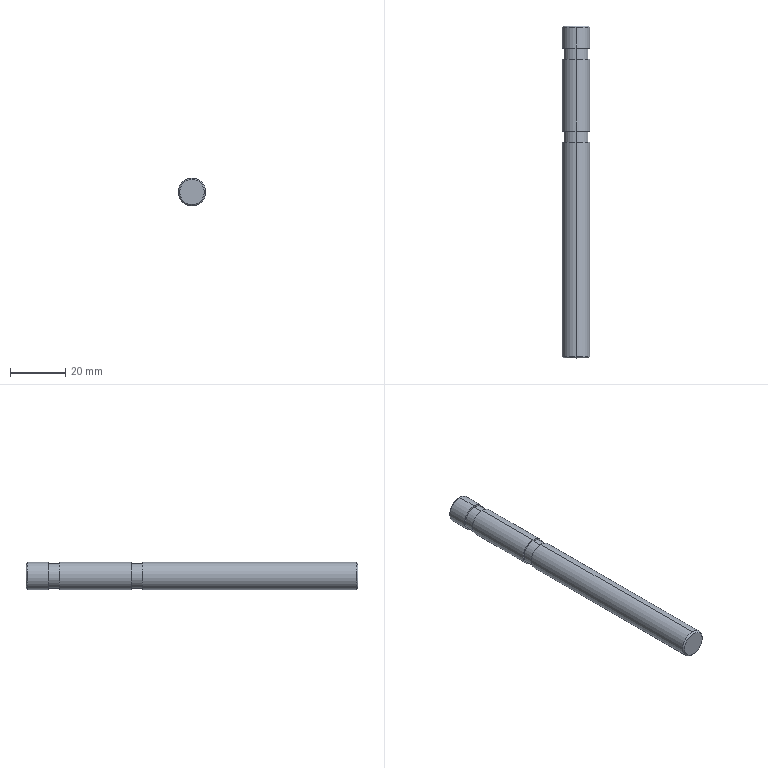Component | SolidWorks | 8TC-A15004-60-30A-2 | 1 solid | 20 faces | box 10 x 120 x 10 mm | volume 9298 mm3 | cylinder 10 | plane 6 | cone 4 | commonest cylinder face diameters 10 x6 9 x4 | material Chrome Plated Hard Rod
build123d program:
from build123d import *

# Parameters (mm, degrees)
SKETCH1_R           = 5
BOSS_EXTRUDE1_DEPTH = 60
CHAMFER1_SIZE       = 0.5
SKETCH2_W           = 1
SKETCH2_H           = 4


with BuildPart() as part:
    # Sketch1 → Boss-Extrude1 (new, symmetric)
    with BuildSketch(Plane(origin=(0, 0, 0), x_dir=(1, 0, 0), z_dir=(0, 1, 0))):
        with Locations(Location((0, 0, 0), (0, 0, 270))):
            Circle(SKETCH1_R)
    extrude(amount=BOSS_EXTRUDE1_DEPTH, both=True)

    # Chamfer1
    chamfer1_edges = [part.edges().sort_by_distance(p)[0] for p in [
        (0, -60, -5),
        (0, 60, -5),
    ]]
    chamfer(chamfer1_edges, length=CHAMFER1_SIZE)

    # Sketch2 → Cut-Revolve1 (revolve, cut)
    with BuildSketch(Plane.XY, mode=Mode.PRIVATE) as cut_revolve1_sk:
        with Locations((5, 50)):
            Rectangle(SKETCH2_W, SKETCH2_H)
        with Locations((5, 20)):
            Rectangle(SKETCH2_W, SKETCH2_H)
    revolve(cut_revolve1_sk.sketch.rotate(Axis((0, 0, 0), (0, -1, 0)), 90), axis=Axis((0, 0, 0), (0, -1, 0)), mode=Mode.SUBTRACT)


solid = part.part

# Placed as in the assembly
solid = solid.moved(Location((-88.286, -35, 0), (0, 0, 0)))
STEP:
#1=COLOUR_RGB('',0.7922,0.8196,0.9333);
#2=FILL_AREA_STYLE_COLOUR('',#1);
#3=FILL_AREA_STYLE('',(#2));
#4=SURFACE_STYLE_FILL_AREA(#3);
#5=SURFACE_SIDE_STYLE('',(#4));
#6=SURFACE_STYLE_USAGE(.BOTH.,#5);
#7=PRESENTATION_STYLE_ASSIGNMENT((#6));
#8=CARTESIAN_POINT('',(-3.476,-0.6693,0.1969));
#9=VERTEX_POINT('',#8);
#10=CARTESIAN_POINT('',(-3.476,-0.6693,-0.1969));
#11=VERTEX_POINT('',#10);
#12=CARTESIAN_POINT('',(-3.476,-0.6693,-0.));
#13=DIRECTION('',(0.,1.,0.));
#14=DIRECTION('',(0.,0.,1.));
#15=AXIS2_PLACEMENT_3D('',#12,#13,#14);
#16=CIRCLE('',#15,0.1969);
#17=EDGE_CURVE('',#9,#11,#16,.T.);
#18=ORIENTED_EDGE('',*,*,#17,.F.);
#19=CARTESIAN_POINT('',(-3.476,-3.72,0.1969));
#20=VERTEX_POINT('',#19);
#21=CARTESIAN_POINT('',(-3.476,0.9843,0.1969));
#22=DIRECTION('',(0.,-1.,0.));
#23=VECTOR('',#22,39.37);
#24=LINE('',#21,#23);
#25=EDGE_CURVE('',#9,#20,#24,.T.);
#26=ORIENTED_EDGE('',*,*,#25,.T.);
#27=CARTESIAN_POINT('',(-3.476,-3.72,-0.1969));
#28=VERTEX_POINT('',#27);
#29=CARTESIAN_POINT('',(-3.476,-3.72,-0.));
#30=DIRECTION('',(0.,1.,0.));
#31=DIRECTION('',(0.,0.,1.));
#32=AXIS2_PLACEMENT_3D('',#29,#30,#31);
#33=CIRCLE('',#32,0.1969);
#34=EDGE_CURVE('',#20,#28,#33,.T.);
#35=ORIENTED_EDGE('',*,*,#34,.T.);
#36=CARTESIAN_POINT('',(-3.476,0.9843,-0.1969));
#37=DIRECTION('',(0.,-1.,0.));
#38=VECTOR('',#37,39.37);
#39=LINE('',#36,#38);
#40=EDGE_CURVE('',#11,#28,#39,.T.);
#41=ORIENTED_EDGE('',*,*,#40,.F.);
#42=EDGE_LOOP('',(#18,#26,#35,#41));
#43=FACE_OUTER_BOUND('',#42,.T.);
#44=CARTESIAN_POINT('',(-3.476,0.9843,-0.));
#45=DIRECTION('',(0.,-1.,0.));
#46=DIRECTION('',(0.,0.,-1.));
#47=AXIS2_PLACEMENT_3D('',#44,#45,#46);
#48=CYLINDRICAL_SURFACE('',#47,0.1969);
#49=ADVANCED_FACE('',(#43),#48,.T.);
#50=CARTESIAN_POINT('',(-3.476,-3.74,-0.1772));
#51=VERTEX_POINT('',#50);
#52=CARTESIAN_POINT('',(-3.476,-3.74,0.1772));
#53=VERTEX_POINT('',#52);
#54=CARTESIAN_POINT('',(-3.476,-3.74,-0.));
#55=DIRECTION('',(0.,-1.,0.));
#56=DIRECTION('',(0.,0.,1.));
#57=AXIS2_PLACEMENT_3D('',#54,#55,#56);
#58=CIRCLE('',#57,0.1772);
#59=EDGE_CURVE('',#51,#53,#58,.T.);
#60=ORIENTED_EDGE('',*,*,#59,.F.);
#61=CARTESIAN_POINT('',(-3.476,-3.72,-0.1969));
#62=DIRECTION('',(0.,0.7071,-0.7071));
#63=VECTOR('',#62,39.37);
#64=LINE('',#61,#63);
#65=EDGE_CURVE('',#51,#28,#64,.T.);
#66=ORIENTED_EDGE('',*,*,#65,.T.);
#67=ORIENTED_EDGE('',*,*,#34,.F.);
#68=CARTESIAN_POINT('',(-3.476,-3.72,0.1969));
#69=DIRECTION('',(0.,0.7071,0.7071));
#70=VECTOR('',#69,39.37);
#71=LINE('',#68,#70);
#72=EDGE_CURVE('',#53,#20,#71,.T.);
#73=ORIENTED_EDGE('',*,*,#72,.F.);
#74=EDGE_LOOP('',(#60,#66,#67,#73));
#75=FACE_OUTER_BOUND('',#74,.T.);
#76=CARTESIAN_POINT('',(-3.476,-3.72,-0.));
#77=DIRECTION('',(0.,1.,0.));
#78=DIRECTION('',(0.,0.,1.));
#79=AXIS2_PLACEMENT_3D('',#76,#77,#78);
#80=CONICAL_SURFACE('',#79,0.1969,0.7854);
#81=ADVANCED_FACE('',(#75),#80,.T.);
#82=CARTESIAN_POINT('',(-3.476,-0.6693,0.1772));
#83=VERTEX_POINT('',#82);
#84=CARTESIAN_POINT('',(-3.476,-0.6693,-0.1772));
#85=VERTEX_POINT('',#84);
#86=CARTESIAN_POINT('',(-3.476,-0.6693,-0.));
#87=DIRECTION('',(0.,1.,0.));
#88=DIRECTION('',(0.,0.,1.));
#89=AXIS2_PLACEMENT_3D('',#86,#87,#88);
#90=CIRCLE('',#89,0.1772);
#91=EDGE_CURVE('',#83,#85,#90,.T.);
#92=ORIENTED_EDGE('',*,*,#91,.T.);
#93=CARTESIAN_POINT('',(-3.476,-0.5118,-0.1772));
#94=VERTEX_POINT('',#93);
#95=CARTESIAN_POINT('',(-3.476,-1.378,-0.1772));
#96=DIRECTION('',(0.,1.,0.));
#97=VECTOR('',#96,39.37);
#98=LINE('',#95,#97);
#99=EDGE_CURVE('',#85,#94,#98,.T.);
#100=ORIENTED_EDGE('',*,*,#99,.T.);
#101=CARTESIAN_POINT('',(-3.476,-0.5118,0.1772));
#102=VERTEX_POINT('',#101);
#103=CARTESIAN_POINT('',(-3.476,-0.5118,-0.));
#104=DIRECTION('',(0.,1.,0.));
#105=DIRECTION('',(0.,0.,1.));
#106=AXIS2_PLACEMENT_3D('',#103,#104,#105);
#107=CIRCLE('',#106,0.1772);
#108=EDGE_CURVE('',#102,#94,#107,.T.);
#109=ORIENTED_EDGE('',*,*,#108,.F.);
#110=CARTESIAN_POINT('',(-3.476,-1.378,0.1772));
#111=DIRECTION('',(0.,1.,0.));
#112=VECTOR('',#111,39.37);
#113=LINE('',#110,#112);
#114=EDGE_CURVE('',#83,#102,#113,.T.);
#115=ORIENTED_EDGE('',*,*,#114,.F.);
#116=EDGE_LOOP('',(#92,#100,#109,#115));
#117=FACE_OUTER_BOUND('',#116,.T.);
#118=CARTESIAN_POINT('',(-3.476,-1.378,-0.));
#119=DIRECTION('',(0.,1.,0.));
#120=DIRECTION('',(0.,0.,1.));
#121=AXIS2_PLACEMENT_3D('',#118,#119,#120);
#122=CYLINDRICAL_SURFACE('',#121,0.1772);
#123=ADVANCED_FACE('',(#117),#122,.T.);
#124=CARTESIAN_POINT('',(-3.476,0.5118,0.1772));
#125=VERTEX_POINT('',#124);
#126=CARTESIAN_POINT('',(-3.476,0.5118,-0.1772));
#127=VERTEX_POINT('',#126);
#128=CARTESIAN_POINT('',(-3.476,0.5118,-0.));
#129=DIRECTION('',(0.,1.,0.));
#130=DIRECTION('',(0.,0.,1.));
#131=AXIS2_PLACEMENT_3D('',#128,#129,#130);
#132=CIRCLE('',#131,0.1772);
#133=EDGE_CURVE('',#125,#127,#132,.T.);
#134=ORIENTED_EDGE('',*,*,#133,.T.);
#135=CARTESIAN_POINT('',(-3.476,0.6693,-0.1772));
#136=VERTEX_POINT('',#135);
#137=CARTESIAN_POINT('',(-3.476,-1.378,-0.1772));
#138=DIRECTION('',(0.,1.,0.));
#139=VECTOR('',#138,39.37);
#140=LINE('',#137,#139);
#141=EDGE_CURVE('',#127,#136,#140,.T.);
#142=ORIENTED_EDGE('',*,*,#141,.T.);
#143=CARTESIAN_POINT('',(-3.476,0.6693,0.1772));
#144=VERTEX_POINT('',#143);
#145=CARTESIAN_POINT('',(-3.476,0.6693,-0.));
#146=DIRECTION('',(0.,1.,0.));
#147=DIRECTION('',(0.,0.,1.));
#148=AXIS2_PLACEMENT_3D('',#145,#146,#147);
#149=CIRCLE('',#148,0.1772);
#150=EDGE_CURVE('',#144,#136,#149,.T.);
#151=ORIENTED_EDGE('',*,*,#150,.F.);
#152=CARTESIAN_POINT('',(-3.476,-1.378,0.1772));
#153=DIRECTION('',(0.,1.,0.));
#154=VECTOR('',#153,39.37);
#155=LINE('',#152,#154);
#156=EDGE_CURVE('',#125,#144,#155,.T.);
#157=ORIENTED_EDGE('',*,*,#156,.F.);
#158=EDGE_LOOP('',(#134,#142,#151,#157));
#159=FACE_OUTER_BOUND('',#158,.T.);
#160=CARTESIAN_POINT('',(-3.476,-1.378,-0.));
#161=DIRECTION('',(0.,1.,0.));
#162=DIRECTION('',(0.,0.,1.));
#163=AXIS2_PLACEMENT_3D('',#160,#161,#162);
#164=CYLINDRICAL_SURFACE('',#163,0.1772);
#165=ADVANCED_FACE('',(#159),#164,.T.);
#166=CARTESIAN_POINT('',(-3.476,0.9843,0.1772));
#167=VERTEX_POINT('',#166);
#168=CARTESIAN_POINT('',(-3.476,0.9843,-0.1772));
#169=VERTEX_POINT('',#168);
#170=CARTESIAN_POINT('',(-3.476,0.9843,-0.));
#171=DIRECTION('',(0.,1.,0.));
#172=DIRECTION('',(0.,0.,1.));
#173=AXIS2_PLACEMENT_3D('',#170,#171,#172);
#174=CIRCLE('',#173,0.1772);
#175=EDGE_CURVE('',#167,#169,#174,.T.);
#176=ORIENTED_EDGE('',*,*,#175,.F.);
#177=CARTESIAN_POINT('',(-3.476,0.9646,0.1969));
#178=VERTEX_POINT('',#177);
#179=CARTESIAN_POINT('',(-3.476,0.9843,0.1772));
#180=DIRECTION('',(0.,-0.7071,0.7071));
#181=VECTOR('',#180,39.37);
#182=LINE('',#179,#181);
#183=EDGE_CURVE('',#167,#178,#182,.T.);
#184=ORIENTED_EDGE('',*,*,#183,.T.);
#185=CARTESIAN_POINT('',(-3.476,0.9646,-0.1969));
#186=VERTEX_POINT('',#185);
#187=CARTESIAN_POINT('',(-3.476,0.9646,-0.));
#188=DIRECTION('',(0.,-1.,0.));
#189=DIRECTION('',(0.,0.,1.));
#190=AXIS2_PLACEMENT_3D('',#187,#188,#189);
#191=CIRCLE('',#190,0.1969);
#192=EDGE_CURVE('',#186,#178,#191,.T.);
#193=ORIENTED_EDGE('',*,*,#192,.F.);
#194=CARTESIAN_POINT('',(-3.476,0.9843,-0.1772));
#195=DIRECTION('',(0.,-0.7071,-0.7071));
#196=VECTOR('',#195,39.37);
#197=LINE('',#194,#196);
#198=EDGE_CURVE('',#169,#186,#197,.T.);
#199=ORIENTED_EDGE('',*,*,#198,.F.);
#200=EDGE_LOOP('',(#176,#184,#193,#199));
#201=FACE_OUTER_BOUND('',#200,.T.);
#202=CARTESIAN_POINT('',(-3.476,0.9843,-0.));
#203=DIRECTION('',(0.,-1.,0.));
#204=DIRECTION('',(0.,0.,-1.));
#205=AXIS2_PLACEMENT_3D('',#202,#203,#204);
#206=CONICAL_SURFACE('',#205,0.1772,0.7854);
#207=ADVANCED_FACE('',(#201),#206,.T.);
#208=ORIENTED_EDGE('',*,*,#192,.T.);
#209=CARTESIAN_POINT('',(-3.476,0.6693,0.1969));
#210=VERTEX_POINT('',#209);
#211=CARTESIAN_POINT('',(-3.476,0.9843,0.1969));
#212=DIRECTION('',(0.,-1.,0.));
#213=VECTOR('',#212,39.37);
#214=LINE('',#211,#213);
#215=EDGE_CURVE('',#178,#210,#214,.T.);
#216=ORIENTED_EDGE('',*,*,#215,.T.);
#217=CARTESIAN_POINT('',(-3.476,0.6693,-0.1969));
#218=VERTEX_POINT('',#217);
#219=CARTESIAN_POINT('',(-3.476,0.6693,-0.));
#220=DIRECTION('',(0.,-1.,0.));
#221=DIRECTION('',(0.,0.,-1.));
#222=AXIS2_PLACEMENT_3D('',#219,#220,#221);
#223=CIRCLE('',#222,0.1969);
#224=EDGE_CURVE('',#218,#210,#223,.T.);
#225=ORIENTED_EDGE('',*,*,#224,.F.);
#226=CARTESIAN_POINT('',(-3.476,0.9843,-0.1969));
#227=DIRECTION('',(0.,-1.,0.));
#228=VECTOR('',#227,39.37);
#229=LINE('',#226,#228);
#230=EDGE_CURVE('',#186,#218,#229,.T.);
#231=ORIENTED_EDGE('',*,*,#230,.F.);
#232=EDGE_LOOP('',(#208,#216,#225,#231));
#233=FACE_OUTER_BOUND('',#232,.T.);
#234=CARTESIAN_POINT('',(-3.476,0.9843,-0.));
#235=DIRECTION('',(0.,-1.,0.));
#236=DIRECTION('',(0.,0.,-1.));
#237=AXIS2_PLACEMENT_3D('',#234,#235,#236);
#238=CYLINDRICAL_SURFACE('',#237,0.1969);
#239=ADVANCED_FACE('',(#233),#238,.T.);
#240=CARTESIAN_POINT('',(-3.476,0.5118,0.1969));
#241=VERTEX_POINT('',#240);
#242=CARTESIAN_POINT('',(-3.476,0.5118,-0.1969));
#243=VERTEX_POINT('',#242);
#244=CARTESIAN_POINT('',(-3.476,0.5118,-0.));
#245=DIRECTION('',(0.,1.,0.));
#246=DIRECTION('',(0.,0.,1.));
#247=AXIS2_PLACEMENT_3D('',#244,#245,#246);
#248=CIRCLE('',#247,0.1969);
#249=EDGE_CURVE('',#241,#243,#248,.T.);
#250=ORIENTED_EDGE('',*,*,#249,.F.);
#251=CARTESIAN_POINT('',(-3.476,-0.5118,0.1969));
#252=VERTEX_POINT('',#251);
#253=CARTESIAN_POINT('',(-3.476,0.9843,0.1969));
#254=DIRECTION('',(0.,-1.,0.));
#255=VECTOR('',#254,39.37);
#256=LINE('',#253,#255);
#257=EDGE_CURVE('',#241,#252,#256,.T.);
#258=ORIENTED_EDGE('',*,*,#257,.T.);
#259=CARTESIAN_POINT('',(-3.476,-0.5118,-0.1969));
#260=VERTEX_POINT('',#259);
#261=CARTESIAN_POINT('',(-3.476,-0.5118,-0.));
#262=DIRECTION('',(0.,-1.,0.));
#263=DIRECTION('',(0.,0.,-1.));
#264=AXIS2_PLACEMENT_3D('',#261,#262,#263);
#265=CIRCLE('',#264,0.1969);
#266=EDGE_CURVE('',#260,#252,#265,.T.);
#267=ORIENTED_EDGE('',*,*,#266,.F.);
#268=CARTESIAN_POINT('',(-3.476,0.9843,-0.1969));
#269=DIRECTION('',(0.,-1.,0.));
#270=VECTOR('',#269,39.37);
#271=LINE('',#268,#270);
#272=EDGE_CURVE('',#243,#260,#271,.T.);
#273=ORIENTED_EDGE('',*,*,#272,.F.);
#274=EDGE_LOOP('',(#250,#258,#267,#273));
#275=FACE_OUTER_BOUND('',#274,.T.);
#276=CARTESIAN_POINT('',(-3.476,0.9843,-0.));
#277=DIRECTION('',(0.,-1.,0.));
#278=DIRECTION('',(0.,0.,-1.));
#279=AXIS2_PLACEMENT_3D('',#276,#277,#278);
#280=CYLINDRICAL_SURFACE('',#279,0.1969);
#281=ADVANCED_FACE('',(#275),#280,.T.);
#282=ORIENTED_EDGE('',*,*,#257,.F.);
#283=CARTESIAN_POINT('',(-3.476,0.5118,-0.));
#284=DIRECTION('',(0.,1.,0.));
#285=DIRECTION('',(0.,0.,1.));
#286=AXIS2_PLACEMENT_3D('',#283,#284,#285);
#287=CIRCLE('',#286,0.1969);
#288=EDGE_CURVE('',#243,#241,#287,.T.);
#289=ORIENTED_EDGE('',*,*,#288,.F.);
#290=ORIENTED_EDGE('',*,*,#272,.T.);
#291=CARTESIAN_POINT('',(-3.476,-0.5118,-0.));
#292=DIRECTION('',(0.,-1.,0.));
#293=DIRECTION('',(0.,0.,-1.));
#294=AXIS2_PLACEMENT_3D('',#291,#292,#293);
#295=CIRCLE('',#294,0.1969);
#296=EDGE_CURVE('',#252,#260,#295,.T.);
#297=ORIENTED_EDGE('',*,*,#296,.F.);
#298=EDGE_LOOP('',(#282,#289,#290,#297));
#299=FACE_OUTER_BOUND('',#298,.T.);
#300=CARTESIAN_POINT('',(-3.476,0.9843,-0.));
#301=DIRECTION('',(0.,-1.,0.));
#302=DIRECTION('',(0.,0.,-1.));
#303=AXIS2_PLACEMENT_3D('',#300,#301,#302);
#304=CYLINDRICAL_SURFACE('',#303,0.1969);
#305=ADVANCED_FACE('',(#299),#304,.T.);
#306=ORIENTED_EDGE('',*,*,#215,.F.);
#307=CARTESIAN_POINT('',(-3.476,0.9646,-0.));
#308=DIRECTION('',(0.,-1.,0.));
#309=DIRECTION('',(0.,0.,1.));
#310=AXIS2_PLACEMENT_3D('',#307,#308,#309);
#311=CIRCLE('',#310,0.1969);
#312=EDGE_CURVE('',#178,#186,#311,.T.);
#313=ORIENTED_EDGE('',*,*,#312,.T.);
#314=ORIENTED_EDGE('',*,*,#230,.T.);
#315=CARTESIAN_POINT('',(-3.476,0.6693,-0.));
#316=DIRECTION('',(0.,-1.,0.));
#317=DIRECTION('',(0.,0.,-1.));
#318=AXIS2_PLACEMENT_3D('',#315,#316,#317);
#319=CIRCLE('',#318,0.1969);
#320=EDGE_CURVE('',#210,#218,#319,.T.);
#321=ORIENTED_EDGE('',*,*,#320,.F.);
#322=EDGE_LOOP('',(#306,#313,#314,#321));
#323=FACE_OUTER_BOUND('',#322,.T.);
#324=CARTESIAN_POINT('',(-3.476,0.9843,-0.));
#325=DIRECTION('',(0.,-1.,0.));
#326=DIRECTION('',(0.,0.,-1.));
#327=AXIS2_PLACEMENT_3D('',#324,#325,#326);
#328=CYLINDRICAL_SURFACE('',#327,0.1969);
#329=ADVANCED_FACE('',(#323),#328,.T.);
#330=CARTESIAN_POINT('',(-3.476,0.9843,-0.));
#331=DIRECTION('',(0.,1.,0.));
#332=DIRECTION('',(0.,0.,1.));
#333=AXIS2_PLACEMENT_3D('',#330,#331,#332);
#334=CIRCLE('',#333,0.1772);
#335=EDGE_CURVE('',#169,#167,#334,.T.);
#336=ORIENTED_EDGE('',*,*,#335,.T.);
#337=ORIENTED_EDGE('',*,*,#175,.T.);
#338=EDGE_LOOP('',(#336,#337));
#339=FACE_OUTER_BOUND('',#338,.T.);
#340=CARTESIAN_POINT('',(-3.476,0.9843,-0.));
#341=DIRECTION('',(0.,1.,0.));
#342=DIRECTION('',(0.,0.,1.));
#343=AXIS2_PLACEMENT_3D('',#340,#341,#342);
#344=PLANE('',#343);
#345=ADVANCED_FACE('',(#339),#344,.T.);
#346=ORIENTED_EDGE('',*,*,#183,.F.);
#347=ORIENTED_EDGE('',*,*,#335,.F.);
#348=ORIENTED_EDGE('',*,*,#198,.T.);
#349=ORIENTED_EDGE('',*,*,#312,.F.);
#350=EDGE_LOOP('',(#346,#347,#348,#349));
#351=FACE_OUTER_BOUND('',#350,.T.);
#352=CARTESIAN_POINT('',(-3.476,0.9843,-0.));
#353=DIRECTION('',(0.,-1.,0.));
#354=DIRECTION('',(0.,0.,-1.));
#355=AXIS2_PLACEMENT_3D('',#352,#353,#354);
#356=CONICAL_SURFACE('',#355,0.1772,0.7854);
#357=ADVANCED_FACE('',(#351),#356,.T.);
#358=ORIENTED_EDGE('',*,*,#150,.T.);
#359=CARTESIAN_POINT('',(-3.476,0.6693,-0.));
#360=DIRECTION('',(0.,1.,0.));
#361=DIRECTION('',(0.,0.,1.));
#362=AXIS2_PLACEMENT_3D('',#359,#360,#361);
#363=CIRCLE('',#362,0.1772);
#364=EDGE_CURVE('',#136,#144,#363,.T.);
#365=ORIENTED_EDGE('',*,*,#364,.T.);
#366=EDGE_LOOP('',(#358,#365));
#367=FACE_BOUND('',#366,.T.);
#368=ORIENTED_EDGE('',*,*,#224,.T.);
#369=ORIENTED_EDGE('',*,*,#320,.T.);
#370=EDGE_LOOP('',(#368,#369));
#371=FACE_OUTER_BOUND('',#370,.T.);
#372=CARTESIAN_POINT('',(-3.259,0.6693,-0.));
#373=DIRECTION('',(0.,-1.,0.));
#374=DIRECTION('',(0.,0.,-1.));
#375=AXIS2_PLACEMENT_3D('',#372,#373,#374);
#376=PLANE('',#375);
#377=ADVANCED_FACE('',(#367,#371),#376,.T.);
#378=ORIENTED_EDGE('',*,*,#133,.F.);
#379=CARTESIAN_POINT('',(-3.476,0.5118,-0.));
#380=DIRECTION('',(0.,1.,0.));
#381=DIRECTION('',(0.,0.,1.));
#382=AXIS2_PLACEMENT_3D('',#379,#380,#381);
#383=CIRCLE('',#382,0.1772);
#384=EDGE_CURVE('',#127,#125,#383,.T.);
#385=ORIENTED_EDGE('',*,*,#384,.F.);
#386=EDGE_LOOP('',(#378,#385));
#387=FACE_BOUND('',#386,.T.);
#388=ORIENTED_EDGE('',*,*,#288,.T.);
#389=ORIENTED_EDGE('',*,*,#249,.T.);
#390=EDGE_LOOP('',(#388,#389));
#391=FACE_OUTER_BOUND('',#390,.T.);
#392=CARTESIAN_POINT('',(-3.259,0.5118,-0.));
#393=DIRECTION('',(0.,1.,0.));
#394=DIRECTION('',(0.,0.,1.));
#395=AXIS2_PLACEMENT_3D('',#392,#393,#394);
#396=PLANE('',#395);
#397=ADVANCED_FACE('',(#387,#391),#396,.T.);
#398=ORIENTED_EDGE('',*,*,#141,.F.);
#399=ORIENTED_EDGE('',*,*,#384,.T.);
#400=ORIENTED_EDGE('',*,*,#156,.T.);
#401=ORIENTED_EDGE('',*,*,#364,.F.);
#402=EDGE_LOOP('',(#398,#399,#400,#401));
#403=FACE_OUTER_BOUND('',#402,.T.);
#404=CARTESIAN_POINT('',(-3.476,-1.378,-0.));
#405=DIRECTION('',(0.,1.,0.));
#406=DIRECTION('',(0.,0.,1.));
#407=AXIS2_PLACEMENT_3D('',#404,#405,#406);
#408=CYLINDRICAL_SURFACE('',#407,0.1772);
#409=ADVANCED_FACE('',(#403),#408,.T.);
#410=ORIENTED_EDGE('',*,*,#108,.T.);
#411=CARTESIAN_POINT('',(-3.476,-0.5118,-0.));
#412=DIRECTION('',(0.,1.,0.));
#413=DIRECTION('',(0.,0.,1.));
#414=AXIS2_PLACEMENT_3D('',#411,#412,#413);
#415=CIRCLE('',#414,0.1772);
#416=EDGE_CURVE('',#94,#102,#415,.T.);
#417=ORIENTED_EDGE('',*,*,#416,.T.);
#418=EDGE_LOOP('',(#410,#417));
#419=FACE_BOUND('',#418,.T.);
#420=ORIENTED_EDGE('',*,*,#266,.T.);
#421=ORIENTED_EDGE('',*,*,#296,.T.);
#422=EDGE_LOOP('',(#420,#421));
#423=FACE_OUTER_BOUND('',#422,.T.);
#424=CARTESIAN_POINT('',(-3.259,-0.5118,-0.));
#425=DIRECTION('',(0.,-1.,0.));
#426=DIRECTION('',(0.,0.,-1.));
#427=AXIS2_PLACEMENT_3D('',#424,#425,#426);
#428=PLANE('',#427);
#429=ADVANCED_FACE('',(#419,#423),#428,.T.);
#430=ORIENTED_EDGE('',*,*,#91,.F.);
#431=CARTESIAN_POINT('',(-3.476,-0.6693,-0.));
#432=DIRECTION('',(0.,1.,0.));
#433=DIRECTION('',(0.,0.,1.));
#434=AXIS2_PLACEMENT_3D('',#431,#432,#433);
#435=CIRCLE('',#434,0.1772);
#436=EDGE_CURVE('',#85,#83,#435,.T.);
#437=ORIENTED_EDGE('',*,*,#436,.F.);
#438=EDGE_LOOP('',(#430,#437));
#439=FACE_BOUND('',#438,.T.);
#440=CARTESIAN_POINT('',(-3.476,-0.6693,-0.));
#441=DIRECTION('',(0.,1.,0.));
#442=DIRECTION('',(0.,0.,1.));
#443=AXIS2_PLACEMENT_3D('',#440,#441,#442);
#444=CIRCLE('',#443,0.1969);
#445=EDGE_CURVE('',#11,#9,#444,.T.);
#446=ORIENTED_EDGE('',*,*,#445,.T.);
#447=ORIENTED_EDGE('',*,*,#17,.T.);
#448=EDGE_LOOP('',(#446,#447));
#449=FACE_OUTER_BOUND('',#448,.T.);
#450=CARTESIAN_POINT('',(-3.259,-0.6693,-0.));
#451=DIRECTION('',(0.,1.,0.));
#452=DIRECTION('',(0.,0.,1.));
#453=AXIS2_PLACEMENT_3D('',#450,#451,#452);
#454=PLANE('',#453);
#455=ADVANCED_FACE('',(#439,#449),#454,.T.);
#456=ORIENTED_EDGE('',*,*,#99,.F.);
#457=ORIENTED_EDGE('',*,*,#436,.T.);
#458=ORIENTED_EDGE('',*,*,#114,.T.);
#459=ORIENTED_EDGE('',*,*,#416,.F.);
#460=EDGE_LOOP('',(#456,#457,#458,#459));
#461=FACE_OUTER_BOUND('',#460,.T.);
#462=CARTESIAN_POINT('',(-3.476,-1.378,-0.));
#463=DIRECTION('',(0.,1.,0.));
#464=DIRECTION('',(0.,0.,1.));
#465=AXIS2_PLACEMENT_3D('',#462,#463,#464);
#466=CYLINDRICAL_SURFACE('',#465,0.1772);
#467=ADVANCED_FACE('',(#461),#466,.T.);
#468=CARTESIAN_POINT('',(-3.476,-3.74,-0.));
#469=DIRECTION('',(0.,-1.,0.));
#470=DIRECTION('',(0.,0.,1.));
#471=AXIS2_PLACEMENT_3D('',#468,#469,#470);
#472=CIRCLE('',#471,0.1772);
#473=EDGE_CURVE('',#53,#51,#472,.T.);
#474=ORIENTED_EDGE('',*,*,#473,.T.);
#475=ORIENTED_EDGE('',*,*,#59,.T.);
#476=EDGE_LOOP('',(#474,#475));
#477=FACE_OUTER_BOUND('',#476,.T.);
#478=CARTESIAN_POINT('',(-3.476,-3.74,-0.));
#479=DIRECTION('',(0.,1.,0.));
#480=DIRECTION('',(0.,0.,1.));
#481=AXIS2_PLACEMENT_3D('',#478,#479,#480);
#482=PLANE('',#481);
#483=ADVANCED_FACE('',(#477),#482,.F.);
#484=ORIENTED_EDGE('',*,*,#65,.F.);
#485=ORIENTED_EDGE('',*,*,#473,.F.);
#486=ORIENTED_EDGE('',*,*,#72,.T.);
#487=CARTESIAN_POINT('',(-3.476,-3.72,-0.));
#488=DIRECTION('',(0.,1.,0.));
#489=DIRECTION('',(0.,0.,1.));
#490=AXIS2_PLACEMENT_3D('',#487,#488,#489);
#491=CIRCLE('',#490,0.1969);
#492=EDGE_CURVE('',#28,#20,#491,.T.);
#493=ORIENTED_EDGE('',*,*,#492,.F.);
#494=EDGE_LOOP('',(#484,#485,#486,#493));
#495=FACE_OUTER_BOUND('',#494,.T.);
#496=CARTESIAN_POINT('',(-3.476,-3.72,-0.));
#497=DIRECTION('',(0.,1.,0.));
#498=DIRECTION('',(0.,0.,1.));
#499=AXIS2_PLACEMENT_3D('',#496,#497,#498);
#500=CONICAL_SURFACE('',#499,0.1969,0.7854);
#501=ADVANCED_FACE('',(#495),#500,.T.);
#502=ORIENTED_EDGE('',*,*,#25,.F.);
#503=ORIENTED_EDGE('',*,*,#445,.F.);
#504=ORIENTED_EDGE('',*,*,#40,.T.);
#505=ORIENTED_EDGE('',*,*,#492,.T.);
#506=EDGE_LOOP('',(#502,#503,#504,#505));
#507=FACE_OUTER_BOUND('',#506,.T.);
#508=CARTESIAN_POINT('',(-3.476,0.9843,-0.));
#509=DIRECTION('',(0.,-1.,0.));
#510=DIRECTION('',(0.,0.,-1.));
#511=AXIS2_PLACEMENT_3D('',#508,#509,#510);
#512=CYLINDRICAL_SURFACE('',#511,0.1969);
#513=ADVANCED_FACE('',(#507),#512,.T.);
#514=CLOSED_SHELL('',(#49,#81,#123,#165,#207,#239,#281,#305,#329,#345,#357,#377,#397,#409,#429,#455,#467,#483,#501,#513));
#515=MANIFOLD_SOLID_BREP('',#514);
#516=STYLED_ITEM('',(#7),#515);
#517=(LENGTH_UNIT()NAMED_UNIT(*)SI_UNIT($,.METRE.));
#518=LENGTH_MEASURE_WITH_UNIT(LENGTH_MEASURE(0.0254),#517);
#519=DIMENSIONAL_EXPONENTS(1.,0.,0.,0.,0.,0.,0.);
#520=(CONVERSION_BASED_UNIT('',#518)LENGTH_UNIT()NAMED_UNIT(#519));
#521=UNCERTAINTY_MEASURE_WITH_UNIT(LENGTH_MEASURE(0.00001),#520,'','');
#522=(NAMED_UNIT(*)PLANE_ANGLE_UNIT()SI_UNIT($,.RADIAN.));
#523=(NAMED_UNIT(*)SI_UNIT($,.STERADIAN.)SOLID_ANGLE_UNIT());
#524=(GEOMETRIC_REPRESENTATION_CONTEXT(3)GLOBAL_UNCERTAINTY_ASSIGNED_CONTEXT((#521))GLOBAL_UNIT_ASSIGNED_CONTEXT((#520,#522,#523))REPRESENTATION_CONTEXT('',''));
#525=MECHANICAL_DESIGN_GEOMETRIC_PRESENTATION_REPRESENTATION('',(#516),#524);
#526=PRESENTATION_LAYER_ASSIGNMENT('','',(#516));
#527=CARTESIAN_POINT('',(0.,0.,0.));
#528=DIRECTION('',(0.,0.,1.));
#529=DIRECTION('',(1.,0.,0.));
#530=AXIS2_PLACEMENT_3D('',#527,#528,#529);
#531=(LENGTH_UNIT()NAMED_UNIT(*)SI_UNIT($,.METRE.));
#532=LENGTH_MEASURE_WITH_UNIT(LENGTH_MEASURE(0.0254),#531);
#533=DIMENSIONAL_EXPONENTS(1.,0.,0.,0.,0.,0.,0.);
#534=(CONVERSION_BASED_UNIT('',#532)LENGTH_UNIT()NAMED_UNIT(#533));
#535=UNCERTAINTY_MEASURE_WITH_UNIT(LENGTH_MEASURE(0.00001),#534,'','');
#536=(NAMED_UNIT(*)PLANE_ANGLE_UNIT()SI_UNIT($,.RADIAN.));
#537=(NAMED_UNIT(*)SI_UNIT($,.STERADIAN.)SOLID_ANGLE_UNIT());
#538=(GEOMETRIC_REPRESENTATION_CONTEXT(3)GLOBAL_UNCERTAINTY_ASSIGNED_CONTEXT((#535))GLOBAL_UNIT_ASSIGNED_CONTEXT((#534,#536,#537))REPRESENTATION_CONTEXT('',''));
#539=ADVANCED_BREP_SHAPE_REPRESENTATION('',(#515,#530),#538);